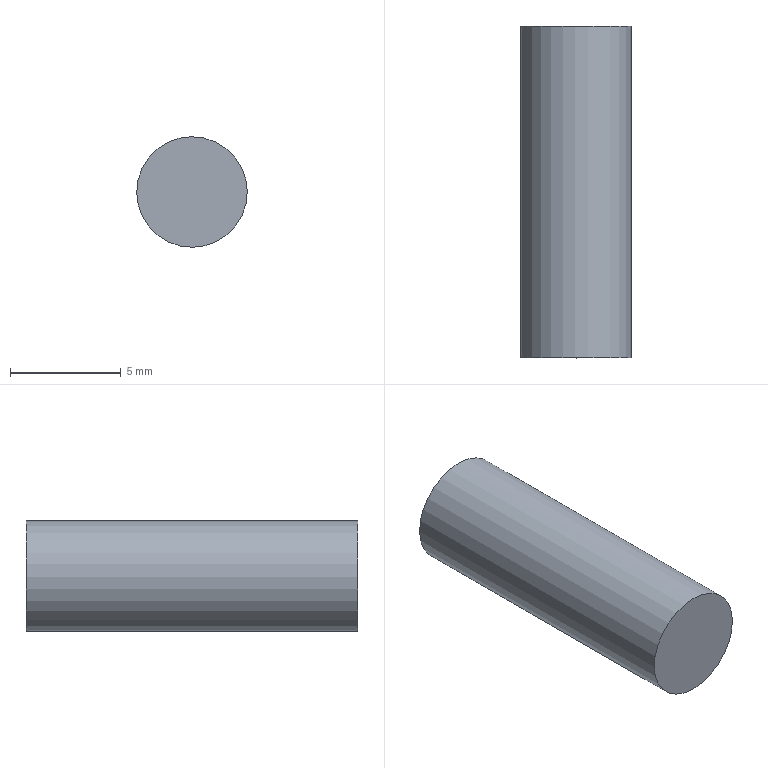Component | NX | CONNECTING_PIN | 1 solid | 3 faces | box 5 x 15 x 5 mm | volume 295 mm3 | plane 2 | cylinder 1 | commonest cylinder face diameters 5 x1
STEP:
#1=CARTESIAN_POINT('',(0.,0.,0.));
#2=DIRECTION('',(0.,0.,1.));
#3=DIRECTION('',(1.,0.,0.));
#4=AXIS2_PLACEMENT_3D('',#1,#2,#3);
#5=CARTESIAN_POINT('',(-29.096,-14.5,16.234));
#6=VERTEX_POINT('',#5);
#7=CARTESIAN_POINT('',(-28.04,-14.5,18.5));
#8=DIRECTION('',(0.,-1.,0.));
#9=DIRECTION('',(-0.4226,0.,-0.9063));
#10=AXIS2_PLACEMENT_3D('',#7,#8,#9);
#11=CIRCLE('',#10,2.5);
#12=CARTESIAN_POINT('',(-28.04,-14.5,18.5));
#13=DIRECTION('',(0.,1.,0.));
#14=DIRECTION('',(-0.4226,0.,-0.9063));
#15=AXIS2_PLACEMENT_3D('',#12,#13,#14);
#16=PLANE('',#15);
#17=CARTESIAN_POINT('',(2.5,0.));
#18=CARTESIAN_POINT('',(2.5,-4.33));
#19=CARTESIAN_POINT('',(-1.25,-2.165));
#20=CARTESIAN_POINT('',(-5.,-0.));
#21=CARTESIAN_POINT('',(-1.25,2.165));
#22=CARTESIAN_POINT('',(2.5,4.33));
#23=CARTESIAN_POINT('',(2.5,0.));
#24=(BOUNDED_CURVE()B_SPLINE_CURVE(2,(#17,#18,#19,#20,#21,#22,#23),.UNSPECIFIED.,.T.,.F.)B_SPLINE_CURVE_WITH_KNOTS((1,2,2,2,2,1),(-2.094,0.,2.094,4.189,6.283,8.378),.UNSPECIFIED.)CURVE()GEOMETRIC_REPRESENTATION_ITEM()RATIONAL_B_SPLINE_CURVE((1.,0.5,1.,0.5,1.,0.5,1.))REPRESENTATION_ITEM(''));
#25=(GEOMETRIC_REPRESENTATION_CONTEXT(2)PARAMETRIC_REPRESENTATION_CONTEXT()REPRESENTATION_CONTEXT('',''));
#26=DEFINITIONAL_REPRESENTATION('',(#24),#25);
#27=PCURVE('',#16,#26);
#28=CARTESIAN_POINT('',(-28.04,-29.5,18.5));
#29=DIRECTION('',(0.,1.,0.));
#30=DIRECTION('',(-0.4226,0.,-0.9063));
#31=AXIS2_PLACEMENT_3D('',#28,#29,#30);
#32=CYLINDRICAL_SURFACE('',#31,2.5);
#33=CARTESIAN_POINT('',(6.283,15.));
#34=DIRECTION('',(-1.,0.));
#35=VECTOR('',#34,1.);
#36=LINE('',#33,#35);
#37=(GEOMETRIC_REPRESENTATION_CONTEXT(2)PARAMETRIC_REPRESENTATION_CONTEXT()REPRESENTATION_CONTEXT('',''));
#38=DEFINITIONAL_REPRESENTATION('',(#36),#37);
#39=PCURVE('',#32,#38);
#40=SURFACE_CURVE('',#11,(#27,#39),.PCURVE_S1.);
#41=EDGE_CURVE('',#6,#6,#40,.T.);
#42=ORIENTED_EDGE('',*,*,#41,.F.);
#43=EDGE_LOOP('',(#42));
#44=FACE_BOUND('',#43,.T.);
#45=ADVANCED_FACE('',(#44),#16,.T.);
#46=CARTESIAN_POINT('',(-29.096,-29.5,16.234));
#47=VERTEX_POINT('',#46);
#48=CARTESIAN_POINT('',(-28.04,-29.5,18.5));
#49=DIRECTION('',(0.,1.,0.));
#50=DIRECTION('',(-0.4226,0.,-0.9063));
#51=AXIS2_PLACEMENT_3D('',#48,#49,#50);
#52=CIRCLE('',#51,2.5);
#53=CARTESIAN_POINT('',(-28.04,-29.5,18.5));
#54=DIRECTION('',(0.,-1.,0.));
#55=DIRECTION('',(0.4226,0.,0.9063));
#56=AXIS2_PLACEMENT_3D('',#53,#54,#55);
#57=PLANE('',#56);
#58=CARTESIAN_POINT('',(-2.5,0.));
#59=CARTESIAN_POINT('',(-2.5,4.33));
#60=CARTESIAN_POINT('',(1.25,2.165));
#61=CARTESIAN_POINT('',(5.,-0.));
#62=CARTESIAN_POINT('',(1.25,-2.165));
#63=CARTESIAN_POINT('',(-2.5,-4.33));
#64=CARTESIAN_POINT('',(-2.5,0.));
#65=(BOUNDED_CURVE()B_SPLINE_CURVE(2,(#58,#59,#60,#61,#62,#63,#64),.UNSPECIFIED.,.T.,.F.)B_SPLINE_CURVE_WITH_KNOTS((1,2,2,2,2,1),(-2.094,0.,2.094,4.189,6.283,8.378),.UNSPECIFIED.)CURVE()GEOMETRIC_REPRESENTATION_ITEM()RATIONAL_B_SPLINE_CURVE((1.,0.5,1.,0.5,1.,0.5,1.))REPRESENTATION_ITEM(''));
#66=(GEOMETRIC_REPRESENTATION_CONTEXT(2)PARAMETRIC_REPRESENTATION_CONTEXT()REPRESENTATION_CONTEXT('',''));
#67=DEFINITIONAL_REPRESENTATION('',(#65),#66);
#68=PCURVE('',#57,#67);
#69=CARTESIAN_POINT('',(0.,0.));
#70=DIRECTION('',(1.,0.));
#71=VECTOR('',#70,1.);
#72=LINE('',#69,#71);
#73=(GEOMETRIC_REPRESENTATION_CONTEXT(2)PARAMETRIC_REPRESENTATION_CONTEXT()REPRESENTATION_CONTEXT('',''));
#74=DEFINITIONAL_REPRESENTATION('',(#72),#73);
#75=PCURVE('',#32,#74);
#76=SURFACE_CURVE('',#52,(#68,#75),.PCURVE_S1.);
#77=EDGE_CURVE('',#47,#47,#76,.T.);
#78=ORIENTED_EDGE('',*,*,#77,.F.);
#79=EDGE_LOOP('',(#78));
#80=FACE_BOUND('',#79,.T.);
#81=ADVANCED_FACE('',(#80),#57,.T.);
#82=ORIENTED_EDGE('',*,*,#41,.T.);
#83=CARTESIAN_POINT('',(-29.096,-29.5,16.234));
#84=CARTESIAN_POINT('',(-29.096,-14.5,16.234));
#85=B_SPLINE_CURVE_WITH_KNOTS('',1,(#83,#84),.UNSPECIFIED.,.F.,.F.,(2,2),(0.,15.),.PIECEWISE_BEZIER_KNOTS.);
#86=CARTESIAN_POINT('',(0.,0.));
#87=DIRECTION('',(0.,1.));
#88=VECTOR('',#87,1.);
#89=LINE('',#86,#88);
#90=(GEOMETRIC_REPRESENTATION_CONTEXT(2)PARAMETRIC_REPRESENTATION_CONTEXT()REPRESENTATION_CONTEXT('',''));
#91=DEFINITIONAL_REPRESENTATION('',(#89),#90);
#92=PCURVE('',#32,#91);
#93=CARTESIAN_POINT('',(6.283,0.));
#94=DIRECTION('',(0.,1.));
#95=VECTOR('',#94,1.);
#96=LINE('',#93,#95);
#97=(GEOMETRIC_REPRESENTATION_CONTEXT(2)PARAMETRIC_REPRESENTATION_CONTEXT()REPRESENTATION_CONTEXT('',''));
#98=DEFINITIONAL_REPRESENTATION('',(#96),#97);
#99=PCURVE('',#32,#98);
#100=SEAM_CURVE('',#85,(#92,#99),.PCURVE_S1.);
#101=EDGE_CURVE('',#47,#6,#100,.T.);
#102=ORIENTED_EDGE('',*,*,#101,.F.);
#103=ORIENTED_EDGE('',*,*,#77,.T.);
#104=ORIENTED_EDGE('',*,*,#101,.T.);
#105=EDGE_LOOP('',(#82,#102,#103,#104));
#106=FACE_BOUND('',#105,.T.);
#107=ADVANCED_FACE('',(#106),#32,.T.);
#108=CLOSED_SHELL('',(#45,#81,#107));
#109=MANIFOLD_SOLID_BREP('',#108);
#110=(LENGTH_UNIT()NAMED_UNIT(*)SI_UNIT(.MILLI.,.METRE.));
#111=UNCERTAINTY_MEASURE_WITH_UNIT(LENGTH_MEASURE(0.00001),#110,'','');
#112=(NAMED_UNIT(*)PLANE_ANGLE_UNIT()SI_UNIT($,.RADIAN.));
#113=(NAMED_UNIT(*)SI_UNIT($,.STERADIAN.)SOLID_ANGLE_UNIT());
#114=(GEOMETRIC_REPRESENTATION_CONTEXT(3)GLOBAL_UNCERTAINTY_ASSIGNED_CONTEXT((#111))GLOBAL_UNIT_ASSIGNED_CONTEXT((#110,#112,#113))REPRESENTATION_CONTEXT('',''));
#115=ADVANCED_BREP_SHAPE_REPRESENTATION('',(#4,#109),#114);